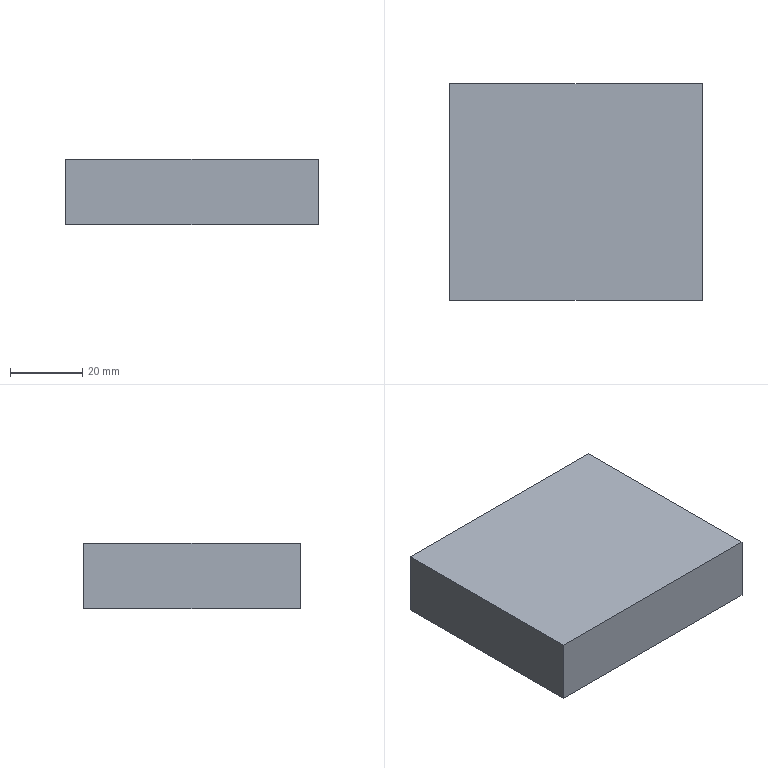Component | NX | SUPPORT_PLATE | 1 solid | 6 faces | box 70 x 60 x 18 mm | volume 75600 mm3 | plane 6
STEP:
#1=CARTESIAN_POINT('',(0.,0.,0.));
#2=DIRECTION('',(0.,0.,1.));
#3=DIRECTION('',(1.,0.,0.));
#4=AXIS2_PLACEMENT_3D('',#1,#2,#3);
#5=CARTESIAN_POINT('',(90.,-30.,80.));
#6=VERTEX_POINT('',#5);
#7=CARTESIAN_POINT('',(20.,-30.,80.));
#8=VERTEX_POINT('',#7);
#9=CARTESIAN_POINT('',(55.,-30.,80.));
#10=DIRECTION('',(-1.,0.,0.));
#11=VECTOR('',#10,1.);
#12=LINE('',#9,#11);
#13=CARTESIAN_POINT('',(55.,-0.,80.));
#14=DIRECTION('',(0.,0.,1.));
#15=DIRECTION('',(1.,0.,0.));
#16=AXIS2_PLACEMENT_3D('',#13,#14,#15);
#17=PLANE('',#16);
#18=CARTESIAN_POINT('',(0.,-30.));
#19=DIRECTION('',(-1.,0.));
#20=VECTOR('',#19,1.);
#21=LINE('',#18,#20);
#22=(GEOMETRIC_REPRESENTATION_CONTEXT(2)PARAMETRIC_REPRESENTATION_CONTEXT()REPRESENTATION_CONTEXT('',''));
#23=DEFINITIONAL_REPRESENTATION('',(#21),#22);
#24=PCURVE('',#17,#23);
#25=CARTESIAN_POINT('',(55.,-30.,62.));
#26=DIRECTION('',(0.,-1.,0.));
#27=DIRECTION('',(0.,0.,-1.));
#28=AXIS2_PLACEMENT_3D('',#25,#26,#27);
#29=PLANE('',#28);
#30=CARTESIAN_POINT('',(-18.,0.));
#31=DIRECTION('',(0.,-1.));
#32=VECTOR('',#31,1.);
#33=LINE('',#30,#32);
#34=(GEOMETRIC_REPRESENTATION_CONTEXT(2)PARAMETRIC_REPRESENTATION_CONTEXT()REPRESENTATION_CONTEXT('',''));
#35=DEFINITIONAL_REPRESENTATION('',(#33),#34);
#36=PCURVE('',#29,#35);
#37=SURFACE_CURVE('',#12,(#24,#36),.PCURVE_S1.);
#38=EDGE_CURVE('',#6,#8,#37,.T.);
#39=ORIENTED_EDGE('',*,*,#38,.F.);
#40=CARTESIAN_POINT('',(90.,30.,80.));
#41=VERTEX_POINT('',#40);
#42=CARTESIAN_POINT('',(90.,-0.,80.));
#43=DIRECTION('',(0.,-1.,0.));
#44=VECTOR('',#43,1.);
#45=LINE('',#42,#44);
#46=CARTESIAN_POINT('',(35.,0.));
#47=DIRECTION('',(0.,-1.));
#48=VECTOR('',#47,1.);
#49=LINE('',#46,#48);
#50=(GEOMETRIC_REPRESENTATION_CONTEXT(2)PARAMETRIC_REPRESENTATION_CONTEXT()REPRESENTATION_CONTEXT('',''));
#51=DEFINITIONAL_REPRESENTATION('',(#49),#50);
#52=PCURVE('',#17,#51);
#53=CARTESIAN_POINT('',(90.,-0.,62.));
#54=DIRECTION('',(1.,0.,0.));
#55=DIRECTION('',(0.,0.,-1.));
#56=AXIS2_PLACEMENT_3D('',#53,#54,#55);
#57=PLANE('',#56);
#58=CARTESIAN_POINT('',(-18.,0.));
#59=DIRECTION('',(0.,-1.));
#60=VECTOR('',#59,1.);
#61=LINE('',#58,#60);
#62=(GEOMETRIC_REPRESENTATION_CONTEXT(2)PARAMETRIC_REPRESENTATION_CONTEXT()REPRESENTATION_CONTEXT('',''));
#63=DEFINITIONAL_REPRESENTATION('',(#61),#62);
#64=PCURVE('',#57,#63);
#65=SURFACE_CURVE('',#45,(#52,#64),.PCURVE_S1.);
#66=EDGE_CURVE('',#41,#6,#65,.T.);
#67=ORIENTED_EDGE('',*,*,#66,.F.);
#68=CARTESIAN_POINT('',(20.,30.,80.));
#69=VERTEX_POINT('',#68);
#70=CARTESIAN_POINT('',(55.,30.,80.));
#71=DIRECTION('',(1.,0.,0.));
#72=VECTOR('',#71,1.);
#73=LINE('',#70,#72);
#74=CARTESIAN_POINT('',(0.,30.));
#75=DIRECTION('',(1.,0.));
#76=VECTOR('',#75,1.);
#77=LINE('',#74,#76);
#78=(GEOMETRIC_REPRESENTATION_CONTEXT(2)PARAMETRIC_REPRESENTATION_CONTEXT()REPRESENTATION_CONTEXT('',''));
#79=DEFINITIONAL_REPRESENTATION('',(#77),#78);
#80=PCURVE('',#17,#79);
#81=CARTESIAN_POINT('',(55.,30.,62.));
#82=DIRECTION('',(0.,1.,0.));
#83=DIRECTION('',(0.,0.,1.));
#84=AXIS2_PLACEMENT_3D('',#81,#82,#83);
#85=PLANE('',#84);
#86=CARTESIAN_POINT('',(18.,0.));
#87=DIRECTION('',(0.,1.));
#88=VECTOR('',#87,1.);
#89=LINE('',#86,#88);
#90=(GEOMETRIC_REPRESENTATION_CONTEXT(2)PARAMETRIC_REPRESENTATION_CONTEXT()REPRESENTATION_CONTEXT('',''));
#91=DEFINITIONAL_REPRESENTATION('',(#89),#90);
#92=PCURVE('',#85,#91);
#93=SURFACE_CURVE('',#73,(#80,#92),.PCURVE_S1.);
#94=EDGE_CURVE('',#69,#41,#93,.T.);
#95=ORIENTED_EDGE('',*,*,#94,.F.);
#96=CARTESIAN_POINT('',(20.,-0.,80.));
#97=DIRECTION('',(0.,1.,0.));
#98=VECTOR('',#97,1.);
#99=LINE('',#96,#98);
#100=CARTESIAN_POINT('',(-35.,0.));
#101=DIRECTION('',(0.,1.));
#102=VECTOR('',#101,1.);
#103=LINE('',#100,#102);
#104=(GEOMETRIC_REPRESENTATION_CONTEXT(2)PARAMETRIC_REPRESENTATION_CONTEXT()REPRESENTATION_CONTEXT('',''));
#105=DEFINITIONAL_REPRESENTATION('',(#103),#104);
#106=PCURVE('',#17,#105);
#107=CARTESIAN_POINT('',(20.,-0.,62.));
#108=DIRECTION('',(-1.,0.,0.));
#109=DIRECTION('',(0.,0.,1.));
#110=AXIS2_PLACEMENT_3D('',#107,#108,#109);
#111=PLANE('',#110);
#112=CARTESIAN_POINT('',(18.,0.));
#113=DIRECTION('',(0.,1.));
#114=VECTOR('',#113,1.);
#115=LINE('',#112,#114);
#116=(GEOMETRIC_REPRESENTATION_CONTEXT(2)PARAMETRIC_REPRESENTATION_CONTEXT()REPRESENTATION_CONTEXT('',''));
#117=DEFINITIONAL_REPRESENTATION('',(#115),#116);
#118=PCURVE('',#111,#117);
#119=SURFACE_CURVE('',#99,(#106,#118),.PCURVE_S1.);
#120=EDGE_CURVE('',#8,#69,#119,.T.);
#121=ORIENTED_EDGE('',*,*,#120,.F.);
#122=EDGE_LOOP('',(#39,#67,#95,#121));
#123=FACE_BOUND('',#122,.T.);
#124=ADVANCED_FACE('',(#123),#17,.T.);
#125=CARTESIAN_POINT('',(90.,-30.,62.));
#126=VERTEX_POINT('',#125);
#127=CARTESIAN_POINT('',(90.,-30.,62.));
#128=DIRECTION('',(0.,0.,1.));
#129=VECTOR('',#128,1.);
#130=LINE('',#127,#129);
#131=CARTESIAN_POINT('',(0.,35.));
#132=DIRECTION('',(-1.,0.));
#133=VECTOR('',#132,1.);
#134=LINE('',#131,#133);
#135=(GEOMETRIC_REPRESENTATION_CONTEXT(2)PARAMETRIC_REPRESENTATION_CONTEXT()REPRESENTATION_CONTEXT('',''));
#136=DEFINITIONAL_REPRESENTATION('',(#134),#135);
#137=PCURVE('',#29,#136);
#138=CARTESIAN_POINT('',(0.,-30.));
#139=DIRECTION('',(-1.,0.));
#140=VECTOR('',#139,1.);
#141=LINE('',#138,#140);
#142=(GEOMETRIC_REPRESENTATION_CONTEXT(2)PARAMETRIC_REPRESENTATION_CONTEXT()REPRESENTATION_CONTEXT('',''));
#143=DEFINITIONAL_REPRESENTATION('',(#141),#142);
#144=PCURVE('',#57,#143);
#145=SURFACE_CURVE('',#130,(#137,#144),.PCURVE_S1.);
#146=EDGE_CURVE('',#126,#6,#145,.T.);
#147=ORIENTED_EDGE('',*,*,#146,.T.);
#148=ORIENTED_EDGE('',*,*,#38,.T.);
#149=CARTESIAN_POINT('',(20.,-30.,62.));
#150=VERTEX_POINT('',#149);
#151=CARTESIAN_POINT('',(20.,-30.,62.));
#152=DIRECTION('',(0.,0.,1.));
#153=VECTOR('',#152,1.);
#154=LINE('',#151,#153);
#155=CARTESIAN_POINT('',(0.,-35.));
#156=DIRECTION('',(-1.,0.));
#157=VECTOR('',#156,1.);
#158=LINE('',#155,#157);
#159=(GEOMETRIC_REPRESENTATION_CONTEXT(2)PARAMETRIC_REPRESENTATION_CONTEXT()REPRESENTATION_CONTEXT('',''));
#160=DEFINITIONAL_REPRESENTATION('',(#158),#159);
#161=PCURVE('',#29,#160);
#162=CARTESIAN_POINT('',(0.,-30.));
#163=DIRECTION('',(1.,0.));
#164=VECTOR('',#163,1.);
#165=LINE('',#162,#164);
#166=(GEOMETRIC_REPRESENTATION_CONTEXT(2)PARAMETRIC_REPRESENTATION_CONTEXT()REPRESENTATION_CONTEXT('',''));
#167=DEFINITIONAL_REPRESENTATION('',(#165),#166);
#168=PCURVE('',#111,#167);
#169=SURFACE_CURVE('',#154,(#161,#168),.PCURVE_S1.);
#170=EDGE_CURVE('',#150,#8,#169,.T.);
#171=ORIENTED_EDGE('',*,*,#170,.F.);
#172=CARTESIAN_POINT('',(55.,-30.,62.));
#173=DIRECTION('',(1.,0.,0.));
#174=VECTOR('',#173,1.);
#175=LINE('',#172,#174);
#176=CARTESIAN_POINT('',(0.,0.));
#177=DIRECTION('',(0.,1.));
#178=VECTOR('',#177,1.);
#179=LINE('',#176,#178);
#180=(GEOMETRIC_REPRESENTATION_CONTEXT(2)PARAMETRIC_REPRESENTATION_CONTEXT()REPRESENTATION_CONTEXT('',''));
#181=DEFINITIONAL_REPRESENTATION('',(#179),#180);
#182=PCURVE('',#29,#181);
#183=CARTESIAN_POINT('',(55.,-0.,62.));
#184=DIRECTION('',(0.,0.,-1.));
#185=DIRECTION('',(-1.,0.,0.));
#186=AXIS2_PLACEMENT_3D('',#183,#184,#185);
#187=PLANE('',#186);
#188=CARTESIAN_POINT('',(0.,-30.));
#189=DIRECTION('',(-1.,0.));
#190=VECTOR('',#189,1.);
#191=LINE('',#188,#190);
#192=(GEOMETRIC_REPRESENTATION_CONTEXT(2)PARAMETRIC_REPRESENTATION_CONTEXT()REPRESENTATION_CONTEXT('',''));
#193=DEFINITIONAL_REPRESENTATION('',(#191),#192);
#194=PCURVE('',#187,#193);
#195=SURFACE_CURVE('',#175,(#182,#194),.PCURVE_S1.);
#196=EDGE_CURVE('',#150,#126,#195,.T.);
#197=ORIENTED_EDGE('',*,*,#196,.T.);
#198=EDGE_LOOP('',(#147,#148,#171,#197));
#199=FACE_BOUND('',#198,.T.);
#200=ADVANCED_FACE('',(#199),#29,.T.);
#201=ORIENTED_EDGE('',*,*,#170,.T.);
#202=ORIENTED_EDGE('',*,*,#120,.T.);
#203=CARTESIAN_POINT('',(20.,30.,62.));
#204=VERTEX_POINT('',#203);
#205=CARTESIAN_POINT('',(20.,30.,62.));
#206=DIRECTION('',(0.,0.,1.));
#207=VECTOR('',#206,1.);
#208=LINE('',#205,#207);
#209=CARTESIAN_POINT('',(0.,30.));
#210=DIRECTION('',(1.,0.));
#211=VECTOR('',#210,1.);
#212=LINE('',#209,#211);
#213=(GEOMETRIC_REPRESENTATION_CONTEXT(2)PARAMETRIC_REPRESENTATION_CONTEXT()REPRESENTATION_CONTEXT('',''));
#214=DEFINITIONAL_REPRESENTATION('',(#212),#213);
#215=PCURVE('',#111,#214);
#216=CARTESIAN_POINT('',(0.,-35.));
#217=DIRECTION('',(1.,0.));
#218=VECTOR('',#217,1.);
#219=LINE('',#216,#218);
#220=(GEOMETRIC_REPRESENTATION_CONTEXT(2)PARAMETRIC_REPRESENTATION_CONTEXT()REPRESENTATION_CONTEXT('',''));
#221=DEFINITIONAL_REPRESENTATION('',(#219),#220);
#222=PCURVE('',#85,#221);
#223=SURFACE_CURVE('',#208,(#215,#222),.PCURVE_S1.);
#224=EDGE_CURVE('',#204,#69,#223,.T.);
#225=ORIENTED_EDGE('',*,*,#224,.F.);
#226=CARTESIAN_POINT('',(20.,-0.,62.));
#227=DIRECTION('',(0.,-1.,0.));
#228=VECTOR('',#227,1.);
#229=LINE('',#226,#228);
#230=CARTESIAN_POINT('',(0.,0.));
#231=DIRECTION('',(0.,-1.));
#232=VECTOR('',#231,1.);
#233=LINE('',#230,#232);
#234=(GEOMETRIC_REPRESENTATION_CONTEXT(2)PARAMETRIC_REPRESENTATION_CONTEXT()REPRESENTATION_CONTEXT('',''));
#235=DEFINITIONAL_REPRESENTATION('',(#233),#234);
#236=PCURVE('',#111,#235);
#237=CARTESIAN_POINT('',(35.,0.));
#238=DIRECTION('',(0.,-1.));
#239=VECTOR('',#238,1.);
#240=LINE('',#237,#239);
#241=(GEOMETRIC_REPRESENTATION_CONTEXT(2)PARAMETRIC_REPRESENTATION_CONTEXT()REPRESENTATION_CONTEXT('',''));
#242=DEFINITIONAL_REPRESENTATION('',(#240),#241);
#243=PCURVE('',#187,#242);
#244=SURFACE_CURVE('',#229,(#236,#243),.PCURVE_S1.);
#245=EDGE_CURVE('',#204,#150,#244,.T.);
#246=ORIENTED_EDGE('',*,*,#245,.T.);
#247=EDGE_LOOP('',(#201,#202,#225,#246));
#248=FACE_BOUND('',#247,.T.);
#249=ADVANCED_FACE('',(#248),#111,.T.);
#250=ORIENTED_EDGE('',*,*,#224,.T.);
#251=ORIENTED_EDGE('',*,*,#94,.T.);
#252=CARTESIAN_POINT('',(90.,30.,62.));
#253=VERTEX_POINT('',#252);
#254=CARTESIAN_POINT('',(90.,30.,62.));
#255=DIRECTION('',(0.,0.,1.));
#256=VECTOR('',#255,1.);
#257=LINE('',#254,#256);
#258=CARTESIAN_POINT('',(0.,35.));
#259=DIRECTION('',(1.,0.));
#260=VECTOR('',#259,1.);
#261=LINE('',#258,#260);
#262=(GEOMETRIC_REPRESENTATION_CONTEXT(2)PARAMETRIC_REPRESENTATION_CONTEXT()REPRESENTATION_CONTEXT('',''));
#263=DEFINITIONAL_REPRESENTATION('',(#261),#262);
#264=PCURVE('',#85,#263);
#265=CARTESIAN_POINT('',(0.,30.));
#266=DIRECTION('',(-1.,0.));
#267=VECTOR('',#266,1.);
#268=LINE('',#265,#267);
#269=(GEOMETRIC_REPRESENTATION_CONTEXT(2)PARAMETRIC_REPRESENTATION_CONTEXT()REPRESENTATION_CONTEXT('',''));
#270=DEFINITIONAL_REPRESENTATION('',(#268),#269);
#271=PCURVE('',#57,#270);
#272=SURFACE_CURVE('',#257,(#264,#271),.PCURVE_S1.);
#273=EDGE_CURVE('',#253,#41,#272,.T.);
#274=ORIENTED_EDGE('',*,*,#273,.F.);
#275=CARTESIAN_POINT('',(55.,30.,62.));
#276=DIRECTION('',(-1.,0.,0.));
#277=VECTOR('',#276,1.);
#278=LINE('',#275,#277);
#279=CARTESIAN_POINT('',(0.,0.));
#280=DIRECTION('',(0.,-1.));
#281=VECTOR('',#280,1.);
#282=LINE('',#279,#281);
#283=(GEOMETRIC_REPRESENTATION_CONTEXT(2)PARAMETRIC_REPRESENTATION_CONTEXT()REPRESENTATION_CONTEXT('',''));
#284=DEFINITIONAL_REPRESENTATION('',(#282),#283);
#285=PCURVE('',#85,#284);
#286=CARTESIAN_POINT('',(0.,30.));
#287=DIRECTION('',(1.,0.));
#288=VECTOR('',#287,1.);
#289=LINE('',#286,#288);
#290=(GEOMETRIC_REPRESENTATION_CONTEXT(2)PARAMETRIC_REPRESENTATION_CONTEXT()REPRESENTATION_CONTEXT('',''));
#291=DEFINITIONAL_REPRESENTATION('',(#289),#290);
#292=PCURVE('',#187,#291);
#293=SURFACE_CURVE('',#278,(#285,#292),.PCURVE_S1.);
#294=EDGE_CURVE('',#253,#204,#293,.T.);
#295=ORIENTED_EDGE('',*,*,#294,.T.);
#296=EDGE_LOOP('',(#250,#251,#274,#295));
#297=FACE_BOUND('',#296,.T.);
#298=ADVANCED_FACE('',(#297),#85,.T.);
#299=CARTESIAN_POINT('',(90.,-0.,62.));
#300=DIRECTION('',(0.,1.,0.));
#301=VECTOR('',#300,1.);
#302=LINE('',#299,#301);
#303=CARTESIAN_POINT('',(-35.,0.));
#304=DIRECTION('',(0.,1.));
#305=VECTOR('',#304,1.);
#306=LINE('',#303,#305);
#307=(GEOMETRIC_REPRESENTATION_CONTEXT(2)PARAMETRIC_REPRESENTATION_CONTEXT()REPRESENTATION_CONTEXT('',''));
#308=DEFINITIONAL_REPRESENTATION('',(#306),#307);
#309=PCURVE('',#187,#308);
#310=CARTESIAN_POINT('',(0.,0.));
#311=DIRECTION('',(0.,1.));
#312=VECTOR('',#311,1.);
#313=LINE('',#310,#312);
#314=(GEOMETRIC_REPRESENTATION_CONTEXT(2)PARAMETRIC_REPRESENTATION_CONTEXT()REPRESENTATION_CONTEXT('',''));
#315=DEFINITIONAL_REPRESENTATION('',(#313),#314);
#316=PCURVE('',#57,#315);
#317=SURFACE_CURVE('',#302,(#309,#316),.PCURVE_S1.);
#318=EDGE_CURVE('',#126,#253,#317,.T.);
#319=ORIENTED_EDGE('',*,*,#318,.F.);
#320=ORIENTED_EDGE('',*,*,#196,.F.);
#321=ORIENTED_EDGE('',*,*,#245,.F.);
#322=ORIENTED_EDGE('',*,*,#294,.F.);
#323=EDGE_LOOP('',(#319,#320,#321,#322));
#324=FACE_BOUND('',#323,.T.);
#325=ADVANCED_FACE('',(#324),#187,.T.);
#326=ORIENTED_EDGE('',*,*,#318,.T.);
#327=ORIENTED_EDGE('',*,*,#273,.T.);
#328=ORIENTED_EDGE('',*,*,#66,.T.);
#329=ORIENTED_EDGE('',*,*,#146,.F.);
#330=EDGE_LOOP('',(#326,#327,#328,#329));
#331=FACE_BOUND('',#330,.T.);
#332=ADVANCED_FACE('',(#331),#57,.T.);
#333=CLOSED_SHELL('',(#124,#200,#249,#298,#325,#332));
#334=MANIFOLD_SOLID_BREP('',#333);
#335=(LENGTH_UNIT()NAMED_UNIT(*)SI_UNIT(.MILLI.,.METRE.));
#336=UNCERTAINTY_MEASURE_WITH_UNIT(LENGTH_MEASURE(0.0000001),#335,'','');
#337=(NAMED_UNIT(*)PLANE_ANGLE_UNIT()SI_UNIT($,.RADIAN.));
#338=(NAMED_UNIT(*)SI_UNIT($,.STERADIAN.)SOLID_ANGLE_UNIT());
#339=(GEOMETRIC_REPRESENTATION_CONTEXT(3)GLOBAL_UNCERTAINTY_ASSIGNED_CONTEXT((#336))GLOBAL_UNIT_ASSIGNED_CONTEXT((#335,#337,#338))REPRESENTATION_CONTEXT('',''));
#340=ADVANCED_BREP_SHAPE_REPRESENTATION('',(#4,#334),#339);